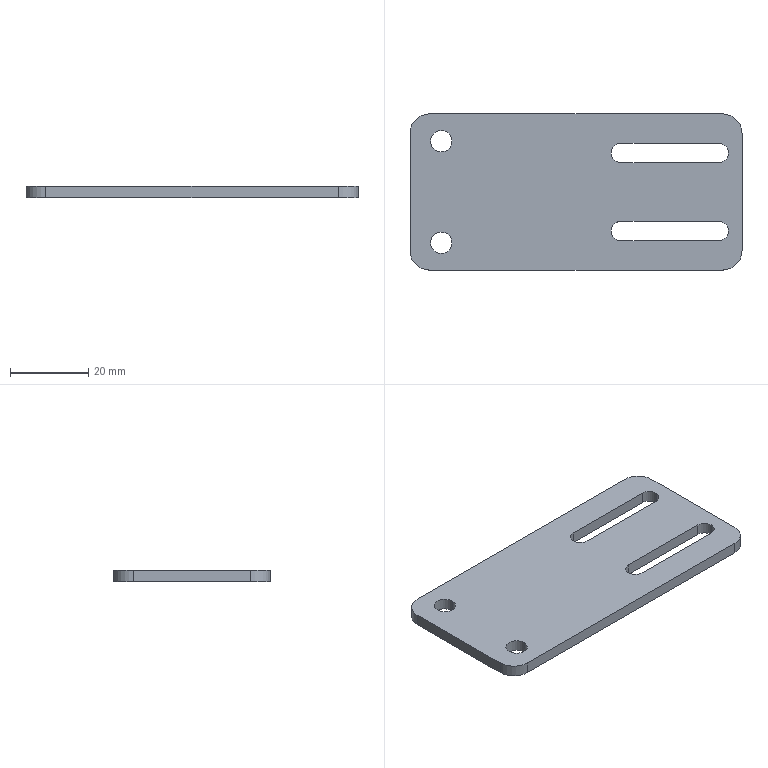Component | SolidWorks | DC-024-43-1 | 1 solid | 24 faces | box 85 x 40 x 3 mm | volume 9125 mm3 | cylinder 14 | plane 10 | commonest cylinder face diameters 5 x6 5.5 x4 10 x4
build123d program:
from build123d import *

# Parameters (mm, degrees)
SKETCH1_W                  = 85
SKETCH1_H                  = 40
BOSS_EXTRUDE1_DEPTH        = 1.5
FILLET1_R                  = 5
F_5_5_5_5_DIAMETER_HOLE1_D = 5.5
CUT_EXTRUDE1_DEPTH         = 20


with BuildPart() as part:
    # Sketch1 → Boss-Extrude1 (new, symmetric)
    with BuildSketch(Plane.XY):
        Rectangle(SKETCH1_W, SKETCH1_H)
    extrude(amount=BOSS_EXTRUDE1_DEPTH, both=True)

    # Fillet1
    fillet1_edges = [part.edges().sort_by_distance(p)[0] for p in [
        (-42.5, 20, 0),
        (42.5, 20, 0),
        (42.5, -20, 0),
        (-42.5, -20, 0),
    ]]
    fillet(fillet1_edges, radius=FILLET1_R)

    # 5.5 _5.5_ Diameter Hole1 (through all)
    with Locations(Plane.XY.offset(1.5)):
        with Locations((-34.5, 13), (-34.5, -13)):
            Hole(F_5_5_5_5_DIAMETER_HOLE1_D / 2)

    # Sketch4 → Cut-Extrude1 (cut)
    with BuildSketch(Plane.XY.offset(1.5)):
        with BuildLine():
            Line((11.5, 12.5), (36.5, 12.5))
            ThreePointArc((36.5, 12.5), (39, 10), (36.5, 7.5))
            Line((36.5, 7.5), (11.5, 7.5))
            ThreePointArc((11.5, 7.5), (9, 10), (11.5, 12.5))
        make_face()
        with BuildLine():
            Line((11.5, -12.5), (36.5, -12.5))
            ThreePointArc((36.5, -12.5), (39, -10), (36.5, -7.5))
            Line((36.5, -7.5), (11.5, -7.5))
            ThreePointArc((11.5, -7.5), (9, -10), (11.5, -12.5))
        make_face()
    extrude(amount=-CUT_EXTRUDE1_DEPTH, mode=Mode.SUBTRACT)


solid = part.part

# Placed as in the assembly
solid = solid.moved(Location((138.867, 171.909, 14.5), (0, 0, 0)))
STEP:
#1=COLOUR_RGB('',0.7922,0.8196,0.9333);
#2=FILL_AREA_STYLE_COLOUR('',#1);
#3=FILL_AREA_STYLE('',(#2));
#4=SURFACE_STYLE_FILL_AREA(#3);
#5=SURFACE_SIDE_STYLE('',(#4));
#6=SURFACE_STYLE_USAGE(.BOTH.,#5);
#7=PRESENTATION_STYLE_ASSIGNMENT((#6));
#8=CARTESIAN_POINT('',(7.003,7.162,0.5118));
#9=VERTEX_POINT('',#8);
#10=CARTESIAN_POINT('',(6.904,7.26,0.5118));
#11=VERTEX_POINT('',#10);
#12=CARTESIAN_POINT('',(6.904,7.162,0.5118));
#13=DIRECTION('',(0.,0.,1.));
#14=DIRECTION('',(1.,0.,0.));
#15=AXIS2_PLACEMENT_3D('',#12,#13,#14);
#16=CIRCLE('',#15,0.09843);
#17=EDGE_CURVE('',#9,#11,#16,.T.);
#18=ORIENTED_EDGE('',*,*,#17,.F.);
#19=CARTESIAN_POINT('',(7.003,7.162,0.6299));
#20=VERTEX_POINT('',#19);
#21=CARTESIAN_POINT('',(7.003,7.162,-0.1575));
#22=DIRECTION('',(0.,0.,1.));
#23=VECTOR('',#22,39.37);
#24=LINE('',#21,#23);
#25=EDGE_CURVE('',#9,#20,#24,.T.);
#26=ORIENTED_EDGE('',*,*,#25,.T.);
#27=CARTESIAN_POINT('',(6.904,7.26,0.6299));
#28=VERTEX_POINT('',#27);
#29=CARTESIAN_POINT('',(6.904,7.162,0.6299));
#30=DIRECTION('',(0.,0.,1.));
#31=DIRECTION('',(1.,0.,0.));
#32=AXIS2_PLACEMENT_3D('',#29,#30,#31);
#33=CIRCLE('',#32,0.09843);
#34=EDGE_CURVE('',#20,#28,#33,.T.);
#35=ORIENTED_EDGE('',*,*,#34,.T.);
#36=CARTESIAN_POINT('',(6.904,7.26,-0.1575));
#37=DIRECTION('',(0.,0.,1.));
#38=VECTOR('',#37,39.37);
#39=LINE('',#36,#38);
#40=EDGE_CURVE('',#11,#28,#39,.T.);
#41=ORIENTED_EDGE('',*,*,#40,.F.);
#42=EDGE_LOOP('',(#18,#26,#35,#41));
#43=FACE_OUTER_BOUND('',#42,.T.);
#44=CARTESIAN_POINT('',(6.904,7.162,-0.1575));
#45=DIRECTION('',(0.,0.,1.));
#46=DIRECTION('',(1.,0.,0.));
#47=AXIS2_PLACEMENT_3D('',#44,#45,#46);
#48=CYLINDRICAL_SURFACE('',#47,0.09843);
#49=ADVANCED_FACE('',(#43),#48,.F.);
#50=CARTESIAN_POINT('',(7.003,6.374,0.5118));
#51=VERTEX_POINT('',#50);
#52=CARTESIAN_POINT('',(6.904,6.473,0.5118));
#53=VERTEX_POINT('',#52);
#54=CARTESIAN_POINT('',(6.904,6.374,0.5118));
#55=DIRECTION('',(0.,0.,1.));
#56=DIRECTION('',(1.,0.,0.));
#57=AXIS2_PLACEMENT_3D('',#54,#55,#56);
#58=CIRCLE('',#57,0.09843);
#59=EDGE_CURVE('',#51,#53,#58,.T.);
#60=ORIENTED_EDGE('',*,*,#59,.F.);
#61=CARTESIAN_POINT('',(7.003,6.374,0.6299));
#62=VERTEX_POINT('',#61);
#63=CARTESIAN_POINT('',(7.003,6.374,-0.1575));
#64=DIRECTION('',(0.,0.,1.));
#65=VECTOR('',#64,39.37);
#66=LINE('',#63,#65);
#67=EDGE_CURVE('',#51,#62,#66,.T.);
#68=ORIENTED_EDGE('',*,*,#67,.T.);
#69=CARTESIAN_POINT('',(6.904,6.473,0.6299));
#70=VERTEX_POINT('',#69);
#71=CARTESIAN_POINT('',(6.904,6.374,0.6299));
#72=DIRECTION('',(0.,0.,1.));
#73=DIRECTION('',(-1.,0.,0.));
#74=AXIS2_PLACEMENT_3D('',#71,#72,#73);
#75=CIRCLE('',#74,0.09843);
#76=EDGE_CURVE('',#62,#70,#75,.T.);
#77=ORIENTED_EDGE('',*,*,#76,.T.);
#78=CARTESIAN_POINT('',(6.904,6.473,-0.1575));
#79=DIRECTION('',(0.,0.,1.));
#80=VECTOR('',#79,39.37);
#81=LINE('',#78,#80);
#82=EDGE_CURVE('',#53,#70,#81,.T.);
#83=ORIENTED_EDGE('',*,*,#82,.F.);
#84=EDGE_LOOP('',(#60,#68,#77,#83));
#85=FACE_OUTER_BOUND('',#84,.T.);
#86=CARTESIAN_POINT('',(6.904,6.374,-0.1575));
#87=DIRECTION('',(0.,0.,1.));
#88=DIRECTION('',(1.,0.,0.));
#89=AXIS2_PLACEMENT_3D('',#86,#87,#88);
#90=CYLINDRICAL_SURFACE('',#89,0.09843);
#91=ADVANCED_FACE('',(#85),#90,.F.);
#92=CARTESIAN_POINT('',(4.001,7.28,0.5118));
#93=VERTEX_POINT('',#92);
#94=CARTESIAN_POINT('',(4.217,7.28,0.5118));
#95=VERTEX_POINT('',#94);
#96=CARTESIAN_POINT('',(4.109,7.28,0.5118));
#97=DIRECTION('',(0.,0.,1.));
#98=DIRECTION('',(1.,0.,0.));
#99=AXIS2_PLACEMENT_3D('',#96,#97,#98);
#100=CIRCLE('',#99,0.1083);
#101=EDGE_CURVE('',#93,#95,#100,.T.);
#102=ORIENTED_EDGE('',*,*,#101,.F.);
#103=CARTESIAN_POINT('',(4.001,7.28,0.6299));
#104=VERTEX_POINT('',#103);
#105=CARTESIAN_POINT('',(4.001,7.28,0.6299));
#106=DIRECTION('',(0.,0.,1.));
#107=VECTOR('',#106,39.37);
#108=LINE('',#105,#107);
#109=EDGE_CURVE('',#93,#104,#108,.T.);
#110=ORIENTED_EDGE('',*,*,#109,.T.);
#111=CARTESIAN_POINT('',(4.217,7.28,0.6299));
#112=VERTEX_POINT('',#111);
#113=CARTESIAN_POINT('',(4.109,7.28,0.6299));
#114=DIRECTION('',(0.,0.,1.));
#115=DIRECTION('',(1.,0.,0.));
#116=AXIS2_PLACEMENT_3D('',#113,#114,#115);
#117=CIRCLE('',#116,0.1083);
#118=EDGE_CURVE('',#104,#112,#117,.T.);
#119=ORIENTED_EDGE('',*,*,#118,.T.);
#120=CARTESIAN_POINT('',(4.217,7.28,0.6299));
#121=DIRECTION('',(0.,0.,1.));
#122=VECTOR('',#121,39.37);
#123=LINE('',#120,#122);
#124=EDGE_CURVE('',#95,#112,#123,.T.);
#125=ORIENTED_EDGE('',*,*,#124,.F.);
#126=EDGE_LOOP('',(#102,#110,#119,#125));
#127=FACE_OUTER_BOUND('',#126,.T.);
#128=CARTESIAN_POINT('',(4.109,7.28,0.6299));
#129=DIRECTION('',(0.,0.,1.));
#130=DIRECTION('',(1.,0.,0.));
#131=AXIS2_PLACEMENT_3D('',#128,#129,#130);
#132=CYLINDRICAL_SURFACE('',#131,0.1083);
#133=ADVANCED_FACE('',(#127),#132,.F.);
#134=CARTESIAN_POINT('',(4.001,6.256,0.5118));
#135=VERTEX_POINT('',#134);
#136=CARTESIAN_POINT('',(4.217,6.256,0.5118));
#137=VERTEX_POINT('',#136);
#138=CARTESIAN_POINT('',(4.109,6.256,0.5118));
#139=DIRECTION('',(0.,0.,1.));
#140=DIRECTION('',(1.,0.,0.));
#141=AXIS2_PLACEMENT_3D('',#138,#139,#140);
#142=CIRCLE('',#141,0.1083);
#143=EDGE_CURVE('',#135,#137,#142,.T.);
#144=ORIENTED_EDGE('',*,*,#143,.F.);
#145=CARTESIAN_POINT('',(4.001,6.256,0.6299));
#146=VERTEX_POINT('',#145);
#147=CARTESIAN_POINT('',(4.001,6.256,0.6299));
#148=DIRECTION('',(0.,0.,1.));
#149=VECTOR('',#148,39.37);
#150=LINE('',#147,#149);
#151=EDGE_CURVE('',#135,#146,#150,.T.);
#152=ORIENTED_EDGE('',*,*,#151,.T.);
#153=CARTESIAN_POINT('',(4.217,6.256,0.6299));
#154=VERTEX_POINT('',#153);
#155=CARTESIAN_POINT('',(4.109,6.256,0.6299));
#156=DIRECTION('',(0.,0.,1.));
#157=DIRECTION('',(1.,0.,0.));
#158=AXIS2_PLACEMENT_3D('',#155,#156,#157);
#159=CIRCLE('',#158,0.1083);
#160=EDGE_CURVE('',#146,#154,#159,.T.);
#161=ORIENTED_EDGE('',*,*,#160,.T.);
#162=CARTESIAN_POINT('',(4.217,6.256,0.6299));
#163=DIRECTION('',(0.,0.,1.));
#164=VECTOR('',#163,39.37);
#165=LINE('',#162,#164);
#166=EDGE_CURVE('',#137,#154,#165,.T.);
#167=ORIENTED_EDGE('',*,*,#166,.F.);
#168=EDGE_LOOP('',(#144,#152,#161,#167));
#169=FACE_OUTER_BOUND('',#168,.T.);
#170=CARTESIAN_POINT('',(4.109,6.256,0.6299));
#171=DIRECTION('',(0.,0.,1.));
#172=DIRECTION('',(1.,0.,0.));
#173=AXIS2_PLACEMENT_3D('',#170,#171,#172);
#174=CYLINDRICAL_SURFACE('',#173,0.1083);
#175=ADVANCED_FACE('',(#169),#174,.F.);
#176=CARTESIAN_POINT('',(3.794,7.359,0.5118));
#177=VERTEX_POINT('',#176);
#178=CARTESIAN_POINT('',(3.794,6.178,0.5118));
#179=VERTEX_POINT('',#178);
#180=CARTESIAN_POINT('',(3.794,5.981,0.5118));
#181=DIRECTION('',(0.,-1.,0.));
#182=VECTOR('',#181,39.37);
#183=LINE('',#180,#182);
#184=EDGE_CURVE('',#177,#179,#183,.T.);
#185=ORIENTED_EDGE('',*,*,#184,.T.);
#186=CARTESIAN_POINT('',(3.794,6.178,0.6299));
#187=VERTEX_POINT('',#186);
#188=CARTESIAN_POINT('',(3.794,6.178,0.6299));
#189=DIRECTION('',(0.,0.,1.));
#190=VECTOR('',#189,39.37);
#191=LINE('',#188,#190);
#192=EDGE_CURVE('',#179,#187,#191,.T.);
#193=ORIENTED_EDGE('',*,*,#192,.T.);
#194=CARTESIAN_POINT('',(3.794,7.359,0.6299));
#195=VERTEX_POINT('',#194);
#196=CARTESIAN_POINT('',(3.794,5.981,0.6299));
#197=DIRECTION('',(0.,-1.,0.));
#198=VECTOR('',#197,39.37);
#199=LINE('',#196,#198);
#200=EDGE_CURVE('',#195,#187,#199,.T.);
#201=ORIENTED_EDGE('',*,*,#200,.F.);
#202=CARTESIAN_POINT('',(3.794,7.359,0.6299));
#203=DIRECTION('',(0.,0.,-1.));
#204=VECTOR('',#203,39.37);
#205=LINE('',#202,#204);
#206=EDGE_CURVE('',#195,#177,#205,.T.);
#207=ORIENTED_EDGE('',*,*,#206,.T.);
#208=EDGE_LOOP('',(#185,#193,#201,#207));
#209=FACE_OUTER_BOUND('',#208,.T.);
#210=CARTESIAN_POINT('',(3.794,5.981,0.6299));
#211=DIRECTION('',(1.,0.,0.));
#212=DIRECTION('',(0.,0.,-1.));
#213=AXIS2_PLACEMENT_3D('',#210,#211,#212);
#214=PLANE('',#213);
#215=ADVANCED_FACE('',(#209),#214,.F.);
#216=CARTESIAN_POINT('',(3.991,5.981,0.5118));
#217=VERTEX_POINT('',#216);
#218=CARTESIAN_POINT('',(6.944,5.981,0.5118));
#219=VERTEX_POINT('',#218);
#220=CARTESIAN_POINT('',(7.14,5.981,0.5118));
#221=DIRECTION('',(1.,0.,0.));
#222=VECTOR('',#221,39.37);
#223=LINE('',#220,#222);
#224=EDGE_CURVE('',#217,#219,#223,.T.);
#225=ORIENTED_EDGE('',*,*,#224,.T.);
#226=CARTESIAN_POINT('',(6.944,5.981,0.6299));
#227=VERTEX_POINT('',#226);
#228=CARTESIAN_POINT('',(6.944,5.981,0.6299));
#229=DIRECTION('',(0.,0.,1.));
#230=VECTOR('',#229,39.37);
#231=LINE('',#228,#230);
#232=EDGE_CURVE('',#219,#227,#231,.T.);
#233=ORIENTED_EDGE('',*,*,#232,.T.);
#234=CARTESIAN_POINT('',(3.991,5.981,0.6299));
#235=VERTEX_POINT('',#234);
#236=CARTESIAN_POINT('',(7.14,5.981,0.6299));
#237=DIRECTION('',(1.,0.,0.));
#238=VECTOR('',#237,39.37);
#239=LINE('',#236,#238);
#240=EDGE_CURVE('',#235,#227,#239,.T.);
#241=ORIENTED_EDGE('',*,*,#240,.F.);
#242=CARTESIAN_POINT('',(3.991,5.981,0.6299));
#243=DIRECTION('',(0.,0.,-1.));
#244=VECTOR('',#243,39.37);
#245=LINE('',#242,#244);
#246=EDGE_CURVE('',#235,#217,#245,.T.);
#247=ORIENTED_EDGE('',*,*,#246,.T.);
#248=EDGE_LOOP('',(#225,#233,#241,#247));
#249=FACE_OUTER_BOUND('',#248,.T.);
#250=CARTESIAN_POINT('',(7.14,5.981,0.6299));
#251=DIRECTION('',(0.,1.,0.));
#252=DIRECTION('',(0.,0.,1.));
#253=AXIS2_PLACEMENT_3D('',#250,#251,#252);
#254=PLANE('',#253);
#255=ADVANCED_FACE('',(#249),#254,.F.);
#256=CARTESIAN_POINT('',(7.14,6.178,0.5118));
#257=VERTEX_POINT('',#256);
#258=CARTESIAN_POINT('',(7.14,7.359,0.5118));
#259=VERTEX_POINT('',#258);
#260=CARTESIAN_POINT('',(7.14,5.981,0.5118));
#261=DIRECTION('',(0.,1.,0.));
#262=VECTOR('',#261,39.37);
#263=LINE('',#260,#262);
#264=EDGE_CURVE('',#257,#259,#263,.T.);
#265=ORIENTED_EDGE('',*,*,#264,.T.);
#266=CARTESIAN_POINT('',(7.14,7.359,0.6299));
#267=VERTEX_POINT('',#266);
#268=CARTESIAN_POINT('',(7.14,7.359,0.6299));
#269=DIRECTION('',(0.,0.,1.));
#270=VECTOR('',#269,39.37);
#271=LINE('',#268,#270);
#272=EDGE_CURVE('',#259,#267,#271,.T.);
#273=ORIENTED_EDGE('',*,*,#272,.T.);
#274=CARTESIAN_POINT('',(7.14,6.178,0.6299));
#275=VERTEX_POINT('',#274);
#276=CARTESIAN_POINT('',(7.14,5.981,0.6299));
#277=DIRECTION('',(0.,1.,0.));
#278=VECTOR('',#277,39.37);
#279=LINE('',#276,#278);
#280=EDGE_CURVE('',#275,#267,#279,.T.);
#281=ORIENTED_EDGE('',*,*,#280,.F.);
#282=CARTESIAN_POINT('',(7.14,6.178,0.6299));
#283=DIRECTION('',(0.,0.,-1.));
#284=VECTOR('',#283,39.37);
#285=LINE('',#282,#284);
#286=EDGE_CURVE('',#275,#257,#285,.T.);
#287=ORIENTED_EDGE('',*,*,#286,.T.);
#288=EDGE_LOOP('',(#265,#273,#281,#287));
#289=FACE_OUTER_BOUND('',#288,.T.);
#290=CARTESIAN_POINT('',(7.14,5.981,0.6299));
#291=DIRECTION('',(-1.,0.,0.));
#292=DIRECTION('',(0.,0.,1.));
#293=AXIS2_PLACEMENT_3D('',#290,#291,#292);
#294=PLANE('',#293);
#295=ADVANCED_FACE('',(#289),#294,.F.);
#296=CARTESIAN_POINT('',(6.944,7.555,0.6299));
#297=VERTEX_POINT('',#296);
#298=CARTESIAN_POINT('',(3.991,7.555,0.6299));
#299=VERTEX_POINT('',#298);
#300=CARTESIAN_POINT('',(7.14,7.555,0.6299));
#301=DIRECTION('',(-1.,0.,0.));
#302=VECTOR('',#301,39.37);
#303=LINE('',#300,#302);
#304=EDGE_CURVE('',#297,#299,#303,.T.);
#305=ORIENTED_EDGE('',*,*,#304,.F.);
#306=CARTESIAN_POINT('',(6.944,7.555,0.5118));
#307=VERTEX_POINT('',#306);
#308=CARTESIAN_POINT('',(6.944,7.555,0.6299));
#309=DIRECTION('',(0.,0.,-1.));
#310=VECTOR('',#309,39.37);
#311=LINE('',#308,#310);
#312=EDGE_CURVE('',#297,#307,#311,.T.);
#313=ORIENTED_EDGE('',*,*,#312,.T.);
#314=CARTESIAN_POINT('',(3.991,7.555,0.5118));
#315=VERTEX_POINT('',#314);
#316=CARTESIAN_POINT('',(7.14,7.555,0.5118));
#317=DIRECTION('',(-1.,0.,0.));
#318=VECTOR('',#317,39.37);
#319=LINE('',#316,#318);
#320=EDGE_CURVE('',#307,#315,#319,.T.);
#321=ORIENTED_EDGE('',*,*,#320,.T.);
#322=CARTESIAN_POINT('',(3.991,7.555,0.6299));
#323=DIRECTION('',(0.,0.,1.));
#324=VECTOR('',#323,39.37);
#325=LINE('',#322,#324);
#326=EDGE_CURVE('',#315,#299,#325,.T.);
#327=ORIENTED_EDGE('',*,*,#326,.T.);
#328=EDGE_LOOP('',(#305,#313,#321,#327));
#329=FACE_OUTER_BOUND('',#328,.T.);
#330=CARTESIAN_POINT('',(7.14,7.555,0.6299));
#331=DIRECTION('',(0.,-1.,0.));
#332=DIRECTION('',(0.,0.,-1.));
#333=AXIS2_PLACEMENT_3D('',#330,#331,#332);
#334=PLANE('',#333);
#335=ADVANCED_FACE('',(#329),#334,.F.);
#336=CARTESIAN_POINT('',(5.92,7.26,0.6299));
#337=VERTEX_POINT('',#336);
#338=CARTESIAN_POINT('',(5.92,7.063,0.6299));
#339=VERTEX_POINT('',#338);
#340=CARTESIAN_POINT('',(5.92,7.162,0.6299));
#341=DIRECTION('',(0.,0.,1.));
#342=DIRECTION('',(1.,0.,0.));
#343=AXIS2_PLACEMENT_3D('',#340,#341,#342);
#344=CIRCLE('',#343,0.09843);
#345=EDGE_CURVE('',#337,#339,#344,.T.);
#346=ORIENTED_EDGE('',*,*,#345,.F.);
#347=CARTESIAN_POINT('',(5.92,7.26,0.6299));
#348=DIRECTION('',(-1.,-0.,0.));
#349=VECTOR('',#348,39.37);
#350=LINE('',#347,#349);
#351=EDGE_CURVE('',#28,#337,#350,.T.);
#352=ORIENTED_EDGE('',*,*,#351,.F.);
#353=ORIENTED_EDGE('',*,*,#34,.F.);
#354=CARTESIAN_POINT('',(6.904,7.063,0.6299));
#355=VERTEX_POINT('',#354);
#356=CARTESIAN_POINT('',(6.904,7.162,0.6299));
#357=DIRECTION('',(0.,0.,1.));
#358=DIRECTION('',(1.,0.,0.));
#359=AXIS2_PLACEMENT_3D('',#356,#357,#358);
#360=CIRCLE('',#359,0.09843);
#361=EDGE_CURVE('',#355,#20,#360,.T.);
#362=ORIENTED_EDGE('',*,*,#361,.F.);
#363=CARTESIAN_POINT('',(5.92,7.063,0.6299));
#364=DIRECTION('',(1.,-0.,0.));
#365=VECTOR('',#364,39.37);
#366=LINE('',#363,#365);
#367=EDGE_CURVE('',#339,#355,#366,.T.);
#368=ORIENTED_EDGE('',*,*,#367,.F.);
#369=EDGE_LOOP('',(#346,#352,#353,#362,#368));
#370=FACE_BOUND('',#369,.T.);
#371=CARTESIAN_POINT('',(5.92,6.473,0.6299));
#372=VERTEX_POINT('',#371);
#373=CARTESIAN_POINT('',(5.92,6.276,0.6299));
#374=VERTEX_POINT('',#373);
#375=CARTESIAN_POINT('',(5.92,6.374,0.6299));
#376=DIRECTION('',(0.,0.,1.));
#377=DIRECTION('',(-1.,0.,0.));
#378=AXIS2_PLACEMENT_3D('',#375,#376,#377);
#379=CIRCLE('',#378,0.09843);
#380=EDGE_CURVE('',#372,#374,#379,.T.);
#381=ORIENTED_EDGE('',*,*,#380,.F.);
#382=CARTESIAN_POINT('',(5.92,6.473,0.6299));
#383=DIRECTION('',(-1.,-0.,0.));
#384=VECTOR('',#383,39.37);
#385=LINE('',#382,#384);
#386=EDGE_CURVE('',#70,#372,#385,.T.);
#387=ORIENTED_EDGE('',*,*,#386,.F.);
#388=ORIENTED_EDGE('',*,*,#76,.F.);
#389=CARTESIAN_POINT('',(6.904,6.276,0.6299));
#390=VERTEX_POINT('',#389);
#391=CARTESIAN_POINT('',(6.904,6.374,0.6299));
#392=DIRECTION('',(0.,0.,1.));
#393=DIRECTION('',(-1.,0.,0.));
#394=AXIS2_PLACEMENT_3D('',#391,#392,#393);
#395=CIRCLE('',#394,0.09843);
#396=EDGE_CURVE('',#390,#62,#395,.T.);
#397=ORIENTED_EDGE('',*,*,#396,.F.);
#398=CARTESIAN_POINT('',(5.92,6.276,0.6299));
#399=DIRECTION('',(1.,-0.,0.));
#400=VECTOR('',#399,39.37);
#401=LINE('',#398,#400);
#402=EDGE_CURVE('',#374,#390,#401,.T.);
#403=ORIENTED_EDGE('',*,*,#402,.F.);
#404=EDGE_LOOP('',(#381,#387,#388,#397,#403));
#405=FACE_BOUND('',#404,.T.);
#406=CARTESIAN_POINT('',(4.109,7.28,0.6299));
#407=DIRECTION('',(0.,0.,1.));
#408=DIRECTION('',(1.,0.,0.));
#409=AXIS2_PLACEMENT_3D('',#406,#407,#408);
#410=CIRCLE('',#409,0.1083);
#411=EDGE_CURVE('',#112,#104,#410,.T.);
#412=ORIENTED_EDGE('',*,*,#411,.F.);
#413=ORIENTED_EDGE('',*,*,#118,.F.);
#414=EDGE_LOOP('',(#412,#413));
#415=FACE_BOUND('',#414,.T.);
#416=CARTESIAN_POINT('',(4.109,6.256,0.6299));
#417=DIRECTION('',(0.,0.,1.));
#418=DIRECTION('',(1.,0.,0.));
#419=AXIS2_PLACEMENT_3D('',#416,#417,#418);
#420=CIRCLE('',#419,0.1083);
#421=EDGE_CURVE('',#154,#146,#420,.T.);
#422=ORIENTED_EDGE('',*,*,#421,.F.);
#423=ORIENTED_EDGE('',*,*,#160,.F.);
#424=EDGE_LOOP('',(#422,#423));
#425=FACE_BOUND('',#424,.T.);
#426=ORIENTED_EDGE('',*,*,#280,.T.);
#427=CARTESIAN_POINT('',(6.944,7.359,0.6299));
#428=DIRECTION('',(0.,0.,1.));
#429=DIRECTION('',(1.,0.,0.));
#430=AXIS2_PLACEMENT_3D('',#427,#428,#429);
#431=CIRCLE('',#430,0.1969);
#432=EDGE_CURVE('',#267,#297,#431,.T.);
#433=ORIENTED_EDGE('',*,*,#432,.T.);
#434=ORIENTED_EDGE('',*,*,#304,.T.);
#435=CARTESIAN_POINT('',(3.991,7.359,0.6299));
#436=DIRECTION('',(0.,0.,1.));
#437=DIRECTION('',(1.,0.,0.));
#438=AXIS2_PLACEMENT_3D('',#435,#436,#437);
#439=CIRCLE('',#438,0.1969);
#440=EDGE_CURVE('',#299,#195,#439,.T.);
#441=ORIENTED_EDGE('',*,*,#440,.T.);
#442=ORIENTED_EDGE('',*,*,#200,.T.);
#443=CARTESIAN_POINT('',(3.991,6.178,0.6299));
#444=DIRECTION('',(0.,0.,1.));
#445=DIRECTION('',(1.,0.,0.));
#446=AXIS2_PLACEMENT_3D('',#443,#444,#445);
#447=CIRCLE('',#446,0.1969);
#448=EDGE_CURVE('',#187,#235,#447,.T.);
#449=ORIENTED_EDGE('',*,*,#448,.T.);
#450=ORIENTED_EDGE('',*,*,#240,.T.);
#451=CARTESIAN_POINT('',(6.944,6.178,0.6299));
#452=DIRECTION('',(0.,0.,1.));
#453=DIRECTION('',(1.,0.,0.));
#454=AXIS2_PLACEMENT_3D('',#451,#452,#453);
#455=CIRCLE('',#454,0.1969);
#456=EDGE_CURVE('',#227,#275,#455,.T.);
#457=ORIENTED_EDGE('',*,*,#456,.T.);
#458=EDGE_LOOP('',(#426,#433,#434,#441,#442,#449,#450,#457));
#459=FACE_OUTER_BOUND('',#458,.T.);
#460=CARTESIAN_POINT('',(5.467,6.768,0.6299));
#461=DIRECTION('',(0.,0.,1.));
#462=DIRECTION('',(1.,0.,0.));
#463=AXIS2_PLACEMENT_3D('',#460,#461,#462);
#464=PLANE('',#463);
#465=ADVANCED_FACE('',(#370,#405,#415,#425,#459),#464,.T.);
#466=CARTESIAN_POINT('',(5.92,7.26,0.5118));
#467=VERTEX_POINT('',#466);
#468=CARTESIAN_POINT('',(5.467,7.26,0.5118));
#469=DIRECTION('',(-1.,-0.,0.));
#470=VECTOR('',#469,39.37);
#471=LINE('',#468,#470);
#472=EDGE_CURVE('',#11,#467,#471,.T.);
#473=ORIENTED_EDGE('',*,*,#472,.T.);
#474=CARTESIAN_POINT('',(5.92,7.063,0.5118));
#475=VERTEX_POINT('',#474);
#476=CARTESIAN_POINT('',(5.92,7.162,0.5118));
#477=DIRECTION('',(0.,0.,1.));
#478=DIRECTION('',(1.,0.,0.));
#479=AXIS2_PLACEMENT_3D('',#476,#477,#478);
#480=CIRCLE('',#479,0.09843);
#481=EDGE_CURVE('',#467,#475,#480,.T.);
#482=ORIENTED_EDGE('',*,*,#481,.T.);
#483=CARTESIAN_POINT('',(6.904,7.063,0.5118));
#484=VERTEX_POINT('',#483);
#485=CARTESIAN_POINT('',(5.467,7.063,0.5118));
#486=DIRECTION('',(1.,-0.,0.));
#487=VECTOR('',#486,39.37);
#488=LINE('',#485,#487);
#489=EDGE_CURVE('',#475,#484,#488,.T.);
#490=ORIENTED_EDGE('',*,*,#489,.T.);
#491=CARTESIAN_POINT('',(6.904,7.162,0.5118));
#492=DIRECTION('',(0.,0.,1.));
#493=DIRECTION('',(1.,0.,0.));
#494=AXIS2_PLACEMENT_3D('',#491,#492,#493);
#495=CIRCLE('',#494,0.09843);
#496=EDGE_CURVE('',#484,#9,#495,.T.);
#497=ORIENTED_EDGE('',*,*,#496,.T.);
#498=ORIENTED_EDGE('',*,*,#17,.T.);
#499=EDGE_LOOP('',(#473,#482,#490,#497,#498));
#500=FACE_BOUND('',#499,.T.);
#501=CARTESIAN_POINT('',(5.92,6.473,0.5118));
#502=VERTEX_POINT('',#501);
#503=CARTESIAN_POINT('',(5.467,6.473,0.5118));
#504=DIRECTION('',(-1.,-0.,0.));
#505=VECTOR('',#504,39.37);
#506=LINE('',#503,#505);
#507=EDGE_CURVE('',#53,#502,#506,.T.);
#508=ORIENTED_EDGE('',*,*,#507,.T.);
#509=CARTESIAN_POINT('',(5.92,6.276,0.5118));
#510=VERTEX_POINT('',#509);
#511=CARTESIAN_POINT('',(5.92,6.374,0.5118));
#512=DIRECTION('',(0.,0.,1.));
#513=DIRECTION('',(1.,0.,0.));
#514=AXIS2_PLACEMENT_3D('',#511,#512,#513);
#515=CIRCLE('',#514,0.09843);
#516=EDGE_CURVE('',#502,#510,#515,.T.);
#517=ORIENTED_EDGE('',*,*,#516,.T.);
#518=CARTESIAN_POINT('',(6.904,6.276,0.5118));
#519=VERTEX_POINT('',#518);
#520=CARTESIAN_POINT('',(5.467,6.276,0.5118));
#521=DIRECTION('',(1.,-0.,0.));
#522=VECTOR('',#521,39.37);
#523=LINE('',#520,#522);
#524=EDGE_CURVE('',#510,#519,#523,.T.);
#525=ORIENTED_EDGE('',*,*,#524,.T.);
#526=CARTESIAN_POINT('',(6.904,6.374,0.5118));
#527=DIRECTION('',(0.,0.,1.));
#528=DIRECTION('',(1.,0.,0.));
#529=AXIS2_PLACEMENT_3D('',#526,#527,#528);
#530=CIRCLE('',#529,0.09843);
#531=EDGE_CURVE('',#519,#51,#530,.T.);
#532=ORIENTED_EDGE('',*,*,#531,.T.);
#533=ORIENTED_EDGE('',*,*,#59,.T.);
#534=EDGE_LOOP('',(#508,#517,#525,#532,#533));
#535=FACE_BOUND('',#534,.T.);
#536=CARTESIAN_POINT('',(4.109,7.28,0.5118));
#537=DIRECTION('',(0.,0.,1.));
#538=DIRECTION('',(1.,0.,0.));
#539=AXIS2_PLACEMENT_3D('',#536,#537,#538);
#540=CIRCLE('',#539,0.1083);
#541=EDGE_CURVE('',#95,#93,#540,.T.);
#542=ORIENTED_EDGE('',*,*,#541,.T.);
#543=ORIENTED_EDGE('',*,*,#101,.T.);
#544=EDGE_LOOP('',(#542,#543));
#545=FACE_BOUND('',#544,.T.);
#546=CARTESIAN_POINT('',(4.109,6.256,0.5118));
#547=DIRECTION('',(0.,0.,1.));
#548=DIRECTION('',(1.,0.,0.));
#549=AXIS2_PLACEMENT_3D('',#546,#547,#548);
#550=CIRCLE('',#549,0.1083);
#551=EDGE_CURVE('',#137,#135,#550,.T.);
#552=ORIENTED_EDGE('',*,*,#551,.T.);
#553=ORIENTED_EDGE('',*,*,#143,.T.);
#554=EDGE_LOOP('',(#552,#553));
#555=FACE_BOUND('',#554,.T.);
#556=ORIENTED_EDGE('',*,*,#320,.F.);
#557=CARTESIAN_POINT('',(6.944,7.359,0.5118));
#558=DIRECTION('',(0.,0.,-1.));
#559=DIRECTION('',(1.,0.,0.));
#560=AXIS2_PLACEMENT_3D('',#557,#558,#559);
#561=CIRCLE('',#560,0.1969);
#562=EDGE_CURVE('',#307,#259,#561,.T.);
#563=ORIENTED_EDGE('',*,*,#562,.T.);
#564=ORIENTED_EDGE('',*,*,#264,.F.);
#565=CARTESIAN_POINT('',(6.944,6.178,0.5118));
#566=DIRECTION('',(0.,0.,-1.));
#567=DIRECTION('',(1.,0.,0.));
#568=AXIS2_PLACEMENT_3D('',#565,#566,#567);
#569=CIRCLE('',#568,0.1969);
#570=EDGE_CURVE('',#257,#219,#569,.T.);
#571=ORIENTED_EDGE('',*,*,#570,.T.);
#572=ORIENTED_EDGE('',*,*,#224,.F.);
#573=CARTESIAN_POINT('',(3.991,6.178,0.5118));
#574=DIRECTION('',(0.,0.,-1.));
#575=DIRECTION('',(1.,0.,0.));
#576=AXIS2_PLACEMENT_3D('',#573,#574,#575);
#577=CIRCLE('',#576,0.1969);
#578=EDGE_CURVE('',#217,#179,#577,.T.);
#579=ORIENTED_EDGE('',*,*,#578,.T.);
#580=ORIENTED_EDGE('',*,*,#184,.F.);
#581=CARTESIAN_POINT('',(3.991,7.359,0.5118));
#582=DIRECTION('',(0.,0.,-1.));
#583=DIRECTION('',(1.,0.,0.));
#584=AXIS2_PLACEMENT_3D('',#581,#582,#583);
#585=CIRCLE('',#584,0.1969);
#586=EDGE_CURVE('',#177,#315,#585,.T.);
#587=ORIENTED_EDGE('',*,*,#586,.T.);
#588=EDGE_LOOP('',(#556,#563,#564,#571,#572,#579,#580,#587));
#589=FACE_OUTER_BOUND('',#588,.T.);
#590=CARTESIAN_POINT('',(5.467,6.768,0.5118));
#591=DIRECTION('',(0.,0.,1.));
#592=DIRECTION('',(1.,0.,0.));
#593=AXIS2_PLACEMENT_3D('',#590,#591,#592);
#594=PLANE('',#593);
#595=ADVANCED_FACE('',(#500,#535,#545,#555,#589),#594,.F.);
#596=ORIENTED_EDGE('',*,*,#432,.F.);
#597=ORIENTED_EDGE('',*,*,#272,.F.);
#598=ORIENTED_EDGE('',*,*,#562,.F.);
#599=ORIENTED_EDGE('',*,*,#312,.F.);
#600=EDGE_LOOP('',(#596,#597,#598,#599));
#601=FACE_OUTER_BOUND('',#600,.T.);
#602=CARTESIAN_POINT('',(6.944,7.359,0.6299));
#603=DIRECTION('',(0.,0.,-1.));
#604=DIRECTION('',(-1.,0.,0.));
#605=AXIS2_PLACEMENT_3D('',#602,#603,#604);
#606=CYLINDRICAL_SURFACE('',#605,0.1969);
#607=ADVANCED_FACE('',(#601),#606,.T.);
#608=ORIENTED_EDGE('',*,*,#456,.F.);
#609=ORIENTED_EDGE('',*,*,#232,.F.);
#610=ORIENTED_EDGE('',*,*,#570,.F.);
#611=ORIENTED_EDGE('',*,*,#286,.F.);
#612=EDGE_LOOP('',(#608,#609,#610,#611));
#613=FACE_OUTER_BOUND('',#612,.T.);
#614=CARTESIAN_POINT('',(6.944,6.178,0.6299));
#615=DIRECTION('',(0.,0.,-1.));
#616=DIRECTION('',(-1.,0.,0.));
#617=AXIS2_PLACEMENT_3D('',#614,#615,#616);
#618=CYLINDRICAL_SURFACE('',#617,0.1969);
#619=ADVANCED_FACE('',(#613),#618,.T.);
#620=ORIENTED_EDGE('',*,*,#448,.F.);
#621=ORIENTED_EDGE('',*,*,#192,.F.);
#622=ORIENTED_EDGE('',*,*,#578,.F.);
#623=ORIENTED_EDGE('',*,*,#246,.F.);
#624=EDGE_LOOP('',(#620,#621,#622,#623));
#625=FACE_OUTER_BOUND('',#624,.T.);
#626=CARTESIAN_POINT('',(3.991,6.178,0.6299));
#627=DIRECTION('',(0.,0.,-1.));
#628=DIRECTION('',(-1.,0.,0.));
#629=AXIS2_PLACEMENT_3D('',#626,#627,#628);
#630=CYLINDRICAL_SURFACE('',#629,0.1969);
#631=ADVANCED_FACE('',(#625),#630,.T.);
#632=ORIENTED_EDGE('',*,*,#440,.F.);
#633=ORIENTED_EDGE('',*,*,#326,.F.);
#634=ORIENTED_EDGE('',*,*,#586,.F.);
#635=ORIENTED_EDGE('',*,*,#206,.F.);
#636=EDGE_LOOP('',(#632,#633,#634,#635));
#637=FACE_OUTER_BOUND('',#636,.T.);
#638=CARTESIAN_POINT('',(3.991,7.359,0.6299));
#639=DIRECTION('',(0.,0.,-1.));
#640=DIRECTION('',(-1.,0.,0.));
#641=AXIS2_PLACEMENT_3D('',#638,#639,#640);
#642=CYLINDRICAL_SURFACE('',#641,0.1969);
#643=ADVANCED_FACE('',(#637),#642,.T.);
#644=ORIENTED_EDGE('',*,*,#151,.F.);
#645=ORIENTED_EDGE('',*,*,#551,.F.);
#646=ORIENTED_EDGE('',*,*,#166,.T.);
#647=ORIENTED_EDGE('',*,*,#421,.T.);
#648=EDGE_LOOP('',(#644,#645,#646,#647));
#649=FACE_OUTER_BOUND('',#648,.T.);
#650=CARTESIAN_POINT('',(4.109,6.256,0.6299));
#651=DIRECTION('',(0.,0.,1.));
#652=DIRECTION('',(1.,0.,0.));
#653=AXIS2_PLACEMENT_3D('',#650,#651,#652);
#654=CYLINDRICAL_SURFACE('',#653,0.1083);
#655=ADVANCED_FACE('',(#649),#654,.F.);
#656=ORIENTED_EDGE('',*,*,#109,.F.);
#657=ORIENTED_EDGE('',*,*,#541,.F.);
#658=ORIENTED_EDGE('',*,*,#124,.T.);
#659=ORIENTED_EDGE('',*,*,#411,.T.);
#660=EDGE_LOOP('',(#656,#657,#658,#659));
#661=FACE_OUTER_BOUND('',#660,.T.);
#662=CARTESIAN_POINT('',(4.109,7.28,0.6299));
#663=DIRECTION('',(0.,0.,1.));
#664=DIRECTION('',(1.,0.,0.));
#665=AXIS2_PLACEMENT_3D('',#662,#663,#664);
#666=CYLINDRICAL_SURFACE('',#665,0.1083);
#667=ADVANCED_FACE('',(#661),#666,.F.);
#668=CARTESIAN_POINT('',(5.92,6.473,-0.1575));
#669=DIRECTION('',(0.,0.,1.));
#670=VECTOR('',#669,39.37);
#671=LINE('',#668,#670);
#672=EDGE_CURVE('',#502,#372,#671,.T.);
#673=ORIENTED_EDGE('',*,*,#672,.T.);
#674=ORIENTED_EDGE('',*,*,#380,.T.);
#675=CARTESIAN_POINT('',(5.92,6.276,-0.1575));
#676=DIRECTION('',(0.,0.,1.));
#677=VECTOR('',#676,39.37);
#678=LINE('',#675,#677);
#679=EDGE_CURVE('',#510,#374,#678,.T.);
#680=ORIENTED_EDGE('',*,*,#679,.F.);
#681=ORIENTED_EDGE('',*,*,#516,.F.);
#682=EDGE_LOOP('',(#673,#674,#680,#681));
#683=FACE_OUTER_BOUND('',#682,.T.);
#684=CARTESIAN_POINT('',(5.92,6.374,-0.1575));
#685=DIRECTION('',(0.,0.,1.));
#686=DIRECTION('',(1.,0.,0.));
#687=AXIS2_PLACEMENT_3D('',#684,#685,#686);
#688=CYLINDRICAL_SURFACE('',#687,0.09843);
#689=ADVANCED_FACE('',(#683),#688,.F.);
#690=ORIENTED_EDGE('',*,*,#82,.T.);
#691=ORIENTED_EDGE('',*,*,#386,.T.);
#692=ORIENTED_EDGE('',*,*,#672,.F.);
#693=ORIENTED_EDGE('',*,*,#507,.F.);
#694=EDGE_LOOP('',(#690,#691,#692,#693));
#695=FACE_OUTER_BOUND('',#694,.T.);
#696=CARTESIAN_POINT('',(5.92,6.473,-0.1575));
#697=DIRECTION('',(-0.,1.,0.));
#698=DIRECTION('',(-1.,-0.,0.));
#699=AXIS2_PLACEMENT_3D('',#696,#697,#698);
#700=PLANE('',#699);
#701=ADVANCED_FACE('',(#695),#700,.F.);
#702=ORIENTED_EDGE('',*,*,#67,.F.);
#703=ORIENTED_EDGE('',*,*,#531,.F.);
#704=CARTESIAN_POINT('',(6.904,6.276,-0.1575));
#705=DIRECTION('',(0.,0.,1.));
#706=VECTOR('',#705,39.37);
#707=LINE('',#704,#706);
#708=EDGE_CURVE('',#519,#390,#707,.T.);
#709=ORIENTED_EDGE('',*,*,#708,.T.);
#710=ORIENTED_EDGE('',*,*,#396,.T.);
#711=EDGE_LOOP('',(#702,#703,#709,#710));
#712=FACE_OUTER_BOUND('',#711,.T.);
#713=CARTESIAN_POINT('',(6.904,6.374,-0.1575));
#714=DIRECTION('',(0.,0.,1.));
#715=DIRECTION('',(1.,0.,0.));
#716=AXIS2_PLACEMENT_3D('',#713,#714,#715);
#717=CYLINDRICAL_SURFACE('',#716,0.09843);
#718=ADVANCED_FACE('',(#712),#717,.F.);
#719=ORIENTED_EDGE('',*,*,#679,.T.);
#720=ORIENTED_EDGE('',*,*,#402,.T.);
#721=ORIENTED_EDGE('',*,*,#708,.F.);
#722=ORIENTED_EDGE('',*,*,#524,.F.);
#723=EDGE_LOOP('',(#719,#720,#721,#722));
#724=FACE_OUTER_BOUND('',#723,.T.);
#725=CARTESIAN_POINT('',(5.92,6.276,-0.1575));
#726=DIRECTION('',(-0.,-1.,0.));
#727=DIRECTION('',(1.,-0.,0.));
#728=AXIS2_PLACEMENT_3D('',#725,#726,#727);
#729=PLANE('',#728);
#730=ADVANCED_FACE('',(#724),#729,.F.);
#731=CARTESIAN_POINT('',(5.92,7.26,-0.1575));
#732=DIRECTION('',(0.,0.,1.));
#733=VECTOR('',#732,39.37);
#734=LINE('',#731,#733);
#735=EDGE_CURVE('',#467,#337,#734,.T.);
#736=ORIENTED_EDGE('',*,*,#735,.T.);
#737=ORIENTED_EDGE('',*,*,#345,.T.);
#738=CARTESIAN_POINT('',(5.92,7.063,-0.1575));
#739=DIRECTION('',(0.,0.,1.));
#740=VECTOR('',#739,39.37);
#741=LINE('',#738,#740);
#742=EDGE_CURVE('',#475,#339,#741,.T.);
#743=ORIENTED_EDGE('',*,*,#742,.F.);
#744=ORIENTED_EDGE('',*,*,#481,.F.);
#745=EDGE_LOOP('',(#736,#737,#743,#744));
#746=FACE_OUTER_BOUND('',#745,.T.);
#747=CARTESIAN_POINT('',(5.92,7.162,-0.1575));
#748=DIRECTION('',(0.,0.,1.));
#749=DIRECTION('',(1.,0.,0.));
#750=AXIS2_PLACEMENT_3D('',#747,#748,#749);
#751=CYLINDRICAL_SURFACE('',#750,0.09843);
#752=ADVANCED_FACE('',(#746),#751,.F.);
#753=ORIENTED_EDGE('',*,*,#40,.T.);
#754=ORIENTED_EDGE('',*,*,#351,.T.);
#755=ORIENTED_EDGE('',*,*,#735,.F.);
#756=ORIENTED_EDGE('',*,*,#472,.F.);
#757=EDGE_LOOP('',(#753,#754,#755,#756));
#758=FACE_OUTER_BOUND('',#757,.T.);
#759=CARTESIAN_POINT('',(5.92,7.26,-0.1575));
#760=DIRECTION('',(-0.,1.,0.));
#761=DIRECTION('',(-1.,-0.,0.));
#762=AXIS2_PLACEMENT_3D('',#759,#760,#761);
#763=PLANE('',#762);
#764=ADVANCED_FACE('',(#758),#763,.F.);
#765=ORIENTED_EDGE('',*,*,#25,.F.);
#766=ORIENTED_EDGE('',*,*,#496,.F.);
#767=CARTESIAN_POINT('',(6.904,7.063,-0.1575));
#768=DIRECTION('',(0.,0.,1.));
#769=VECTOR('',#768,39.37);
#770=LINE('',#767,#769);
#771=EDGE_CURVE('',#484,#355,#770,.T.);
#772=ORIENTED_EDGE('',*,*,#771,.T.);
#773=ORIENTED_EDGE('',*,*,#361,.T.);
#774=EDGE_LOOP('',(#765,#766,#772,#773));
#775=FACE_OUTER_BOUND('',#774,.T.);
#776=CARTESIAN_POINT('',(6.904,7.162,-0.1575));
#777=DIRECTION('',(0.,0.,1.));
#778=DIRECTION('',(1.,0.,0.));
#779=AXIS2_PLACEMENT_3D('',#776,#777,#778);
#780=CYLINDRICAL_SURFACE('',#779,0.09843);
#781=ADVANCED_FACE('',(#775),#780,.F.);
#782=ORIENTED_EDGE('',*,*,#742,.T.);
#783=ORIENTED_EDGE('',*,*,#367,.T.);
#784=ORIENTED_EDGE('',*,*,#771,.F.);
#785=ORIENTED_EDGE('',*,*,#489,.F.);
#786=EDGE_LOOP('',(#782,#783,#784,#785));
#787=FACE_OUTER_BOUND('',#786,.T.);
#788=CARTESIAN_POINT('',(5.92,7.063,-0.1575));
#789=DIRECTION('',(-0.,-1.,0.));
#790=DIRECTION('',(1.,-0.,0.));
#791=AXIS2_PLACEMENT_3D('',#788,#789,#790);
#792=PLANE('',#791);
#793=ADVANCED_FACE('',(#787),#792,.F.);
#794=CLOSED_SHELL('',(#49,#91,#133,#175,#215,#255,#295,#335,#465,#595,#607,#619,#631,#643,#655,#667,#689,#701,#718,#730,#752,#764,#781,#793));
#795=MANIFOLD_SOLID_BREP('',#794);
#796=STYLED_ITEM('',(#7),#795);
#797=PRESENTATION_LAYER_ASSIGNMENT('','',(#796));
#798=CARTESIAN_POINT('',(0.,0.,0.));
#799=DIRECTION('',(0.,0.,1.));
#800=DIRECTION('',(1.,0.,0.));
#801=AXIS2_PLACEMENT_3D('',#798,#799,#800);
#802=(LENGTH_UNIT()NAMED_UNIT(*)SI_UNIT($,.METRE.));
#803=LENGTH_MEASURE_WITH_UNIT(LENGTH_MEASURE(0.0254),#802);
#804=DIMENSIONAL_EXPONENTS(1.,0.,0.,0.,0.,0.,0.);
#805=(CONVERSION_BASED_UNIT('',#803)LENGTH_UNIT()NAMED_UNIT(#804));
#806=UNCERTAINTY_MEASURE_WITH_UNIT(LENGTH_MEASURE(0.00001),#805,'','');
#807=(NAMED_UNIT(*)PLANE_ANGLE_UNIT()SI_UNIT($,.RADIAN.));
#808=(NAMED_UNIT(*)SI_UNIT($,.STERADIAN.)SOLID_ANGLE_UNIT());
#809=(GEOMETRIC_REPRESENTATION_CONTEXT(3)GLOBAL_UNCERTAINTY_ASSIGNED_CONTEXT((#806))GLOBAL_UNIT_ASSIGNED_CONTEXT((#805,#807,#808))REPRESENTATION_CONTEXT('',''));
#810=ADVANCED_BREP_SHAPE_REPRESENTATION('',(#795,#801),#809);
#811=(LENGTH_UNIT()NAMED_UNIT(*)SI_UNIT($,.METRE.));
#812=LENGTH_MEASURE_WITH_UNIT(LENGTH_MEASURE(0.0254),#811);
#813=DIMENSIONAL_EXPONENTS(1.,0.,0.,0.,0.,0.,0.);
#814=(CONVERSION_BASED_UNIT('',#812)LENGTH_UNIT()NAMED_UNIT(#813));
#815=UNCERTAINTY_MEASURE_WITH_UNIT(LENGTH_MEASURE(0.00001),#814,'','');
#816=(NAMED_UNIT(*)PLANE_ANGLE_UNIT()SI_UNIT($,.RADIAN.));
#817=(NAMED_UNIT(*)SI_UNIT($,.STERADIAN.)SOLID_ANGLE_UNIT());
#818=(GEOMETRIC_REPRESENTATION_CONTEXT(3)GLOBAL_UNCERTAINTY_ASSIGNED_CONTEXT((#815))GLOBAL_UNIT_ASSIGNED_CONTEXT((#814,#816,#817))REPRESENTATION_CONTEXT('',''));
#819=MECHANICAL_DESIGN_GEOMETRIC_PRESENTATION_REPRESENTATION('',(#796),#818);